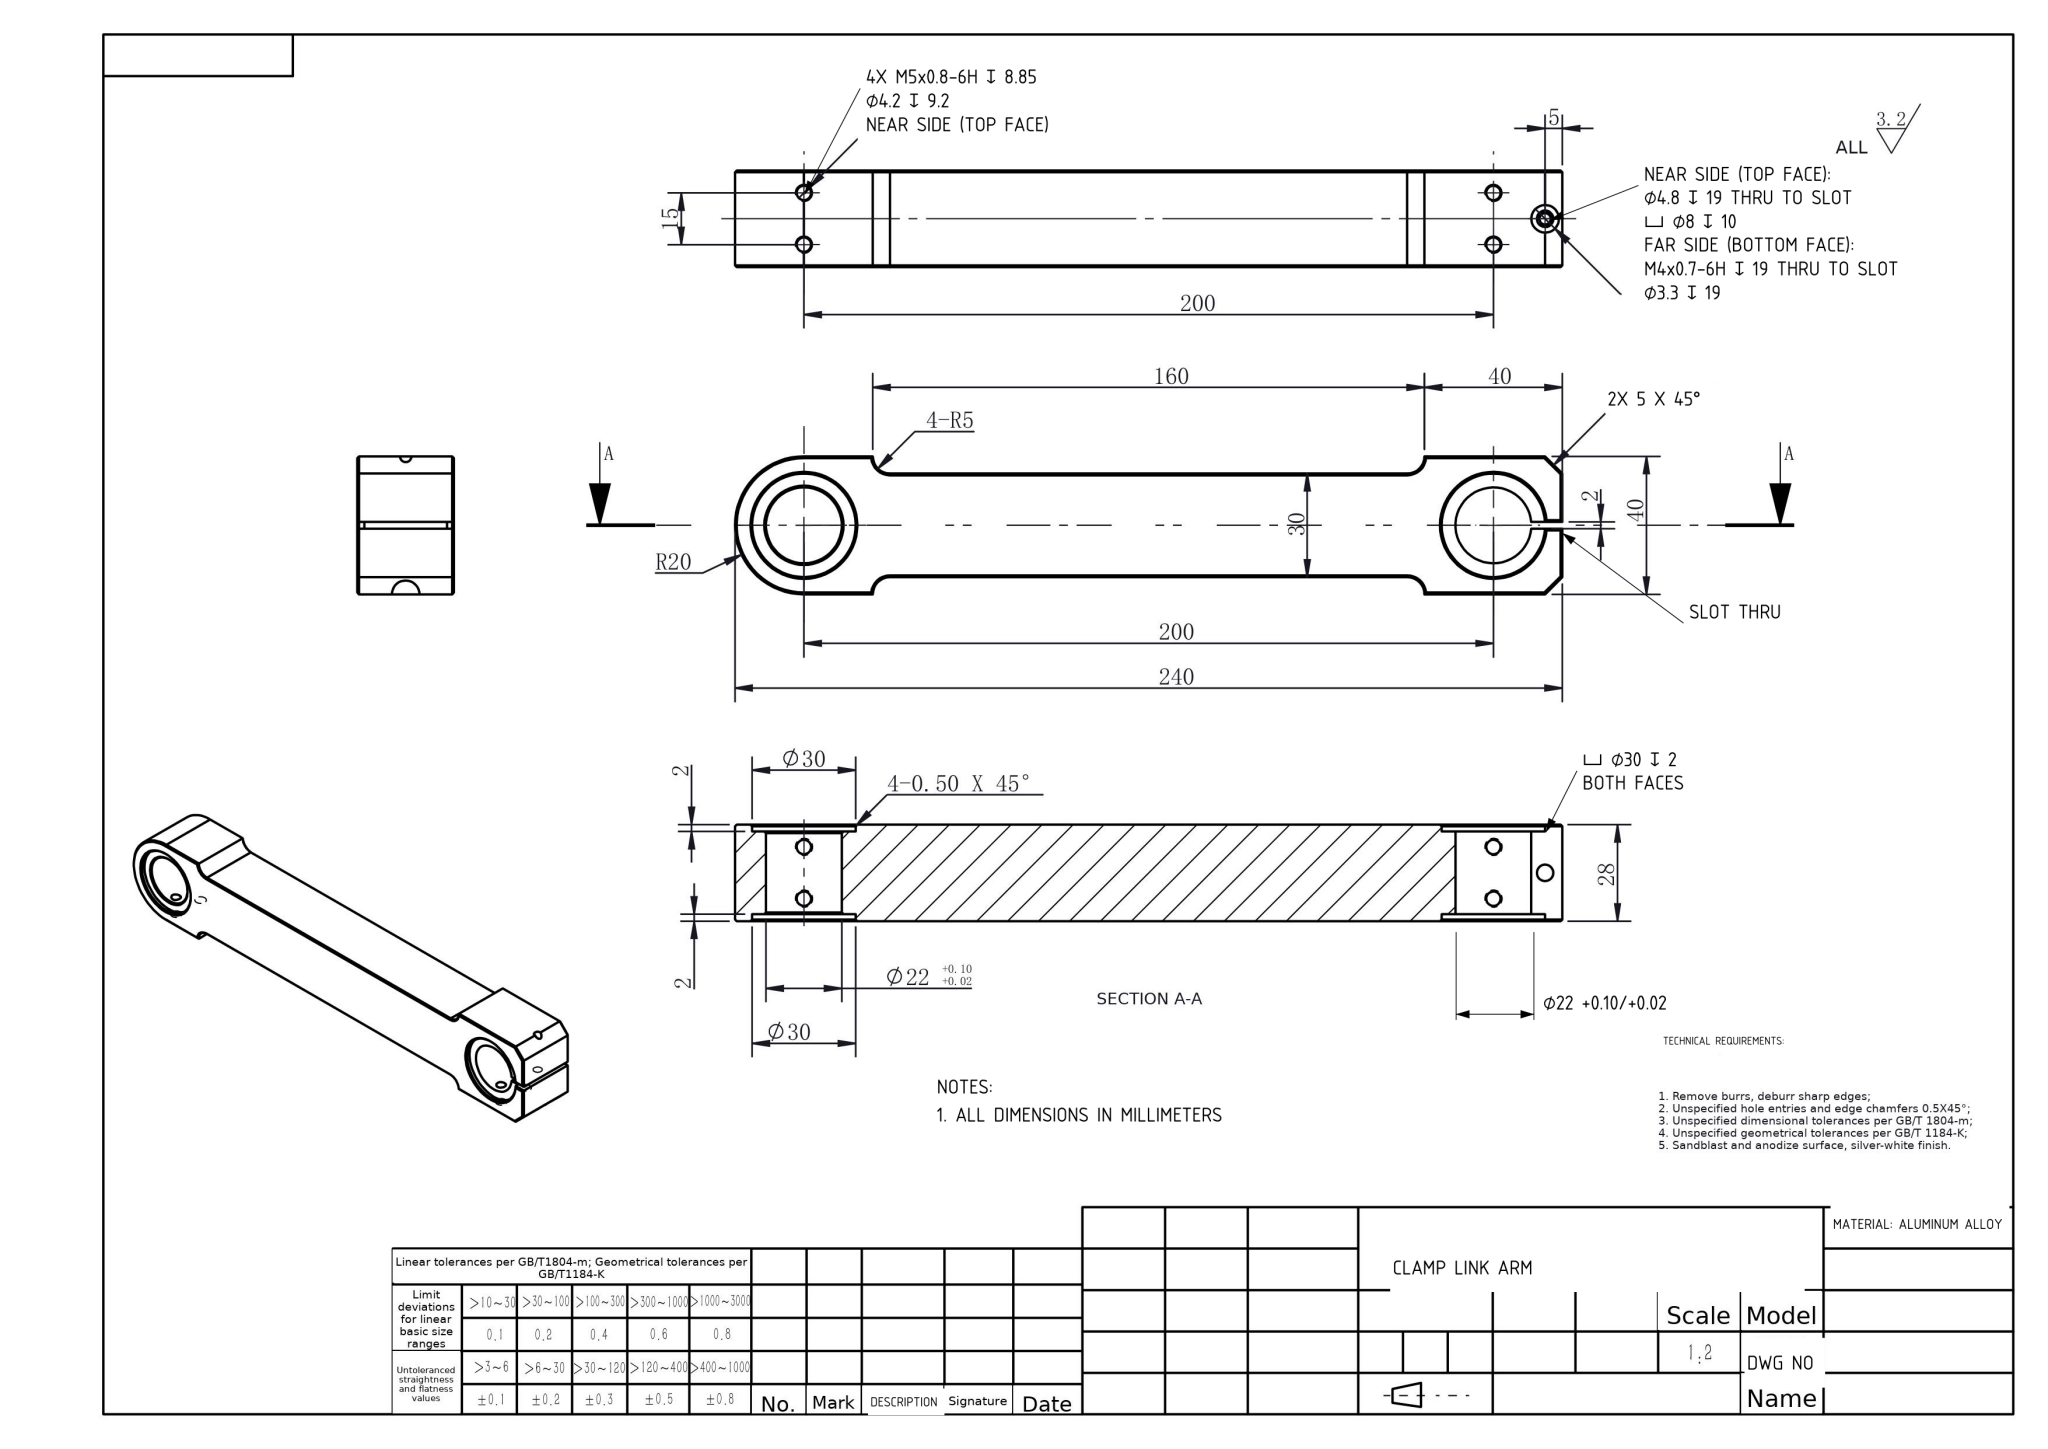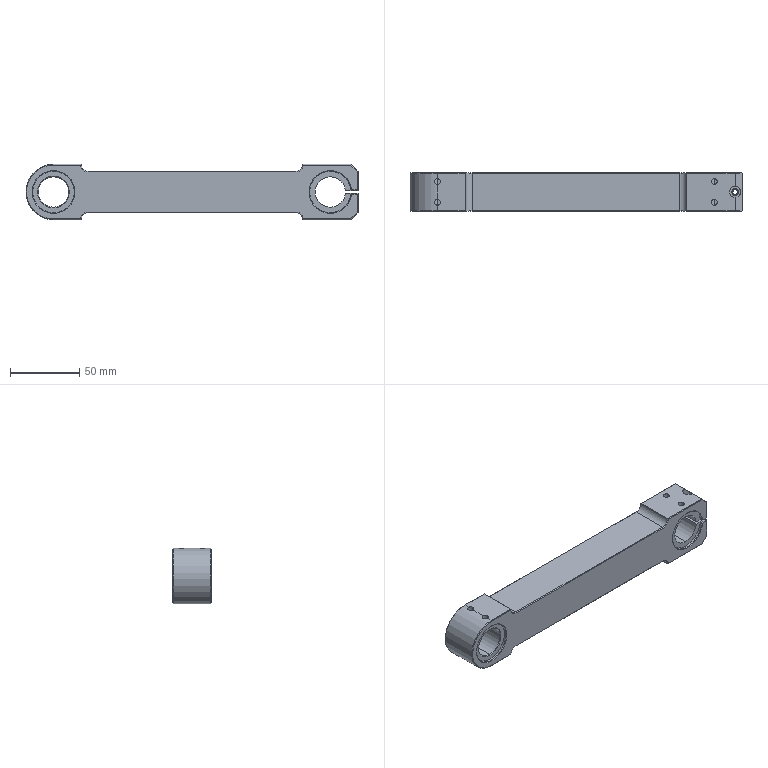Part | NX | mm | 1 solid | 101 faces | box 240 x 28 x 40 mm | volume 193233 mm3 | plane 43 | cylinder 34 | cone 24 | commonest cylinder face diameters 30 x10 4.2 x8 22 x5 10 x4 3.3 x2 8 x2 4.8 x2 40 x1